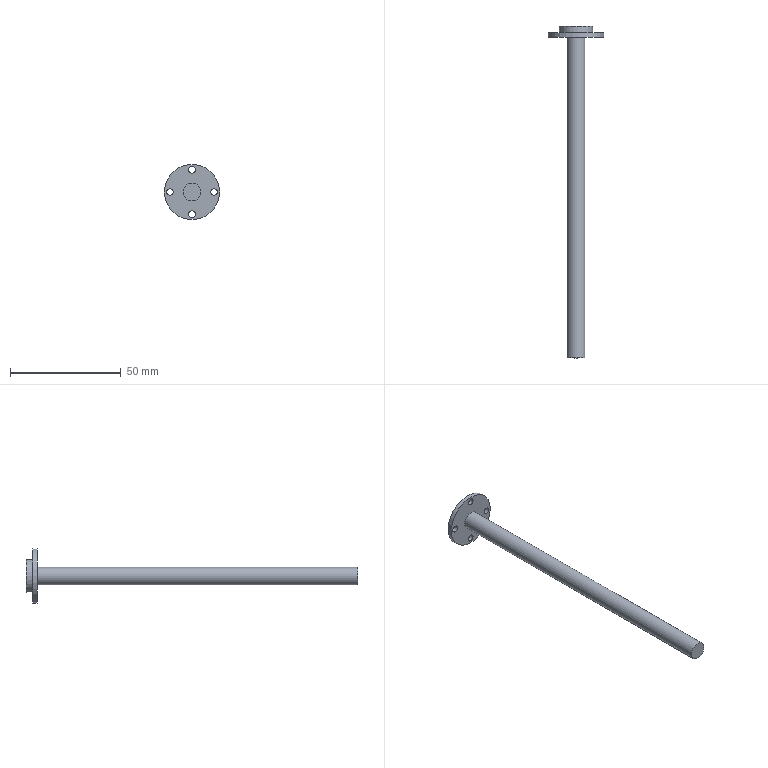Component | NX | GEAR_SHAFT_2 | 1 solid | 11 faces | box 25 x 150 x 25 mm | volume 8744 mm3 | cylinder 7 | plane 4 | commonest cylinder face diameters 3 x4 8 x1 25 x1 15 x1
STEP:
#1=CARTESIAN_POINT('',(0.,0.,0.));
#2=DIRECTION('',(0.,0.,1.));
#3=DIRECTION('',(1.,0.,0.));
#4=AXIS2_PLACEMENT_3D('',#1,#2,#3);
#5=CARTESIAN_POINT('',(-129.451,-34.96,29.835));
#6=VERTEX_POINT('',#5);
#7=CARTESIAN_POINT('',(-133.451,-34.96,29.835));
#8=DIRECTION('',(0.,1.,0.));
#9=DIRECTION('',(1.,0.,0.));
#10=AXIS2_PLACEMENT_3D('',#7,#8,#9);
#11=CIRCLE('',#10,4.);
#12=CARTESIAN_POINT('',(-133.451,-34.96,29.835));
#13=DIRECTION('',(0.,1.,0.));
#14=DIRECTION('',(0.,0.,1.));
#15=AXIS2_PLACEMENT_3D('',#12,#13,#14);
#16=CYLINDRICAL_SURFACE('',#15,4.);
#17=CARTESIAN_POINT('',(1.571,0.));
#18=DIRECTION('',(1.,0.));
#19=VECTOR('',#18,1.);
#20=LINE('',#17,#19);
#21=(GEOMETRIC_REPRESENTATION_CONTEXT(2)PARAMETRIC_REPRESENTATION_CONTEXT()REPRESENTATION_CONTEXT('',''));
#22=DEFINITIONAL_REPRESENTATION('',(#20),#21);
#23=PCURVE('',#16,#22);
#24=CARTESIAN_POINT('',(-133.451,-34.96,29.835));
#25=DIRECTION('',(0.,1.,0.));
#26=DIRECTION('',(0.,0.,1.));
#27=AXIS2_PLACEMENT_3D('',#24,#25,#26);
#28=PLANE('',#27);
#29=CARTESIAN_POINT('',(0.,0.));
#30=DIRECTION('',(0.,1.));
#31=AXIS2_PLACEMENT_2D('',#29,#30);
#32=CIRCLE('',#31,4.);
#33=(GEOMETRIC_REPRESENTATION_CONTEXT(2)PARAMETRIC_REPRESENTATION_CONTEXT()REPRESENTATION_CONTEXT('',''));
#34=DEFINITIONAL_REPRESENTATION('',(#32),#33);
#35=PCURVE('',#28,#34);
#36=SURFACE_CURVE('',#11,(#23,#35),.PCURVE_S1.);
#37=EDGE_CURVE('',#6,#6,#36,.T.);
#38=ORIENTED_EDGE('',*,*,#37,.T.);
#39=CARTESIAN_POINT('',(-129.451,110.04,29.835));
#40=VERTEX_POINT('',#39);
#41=CARTESIAN_POINT('',(-129.451,-34.96,29.835));
#42=CARTESIAN_POINT('',(-129.451,110.04,29.835));
#43=B_SPLINE_CURVE_WITH_KNOTS('',1,(#41,#42),.UNSPECIFIED.,.F.,.F.,(2,2),(0.,145.),.PIECEWISE_BEZIER_KNOTS.);
#44=CARTESIAN_POINT('',(7.854,0.));
#45=DIRECTION('',(0.,1.));
#46=VECTOR('',#45,1.);
#47=LINE('',#44,#46);
#48=(GEOMETRIC_REPRESENTATION_CONTEXT(2)PARAMETRIC_REPRESENTATION_CONTEXT()REPRESENTATION_CONTEXT('',''));
#49=DEFINITIONAL_REPRESENTATION('',(#47),#48);
#50=PCURVE('',#16,#49);
#51=CARTESIAN_POINT('',(1.571,0.));
#52=DIRECTION('',(0.,1.));
#53=VECTOR('',#52,1.);
#54=LINE('',#51,#53);
#55=(GEOMETRIC_REPRESENTATION_CONTEXT(2)PARAMETRIC_REPRESENTATION_CONTEXT()REPRESENTATION_CONTEXT('',''));
#56=DEFINITIONAL_REPRESENTATION('',(#54),#55);
#57=PCURVE('',#16,#56);
#58=SEAM_CURVE('',#43,(#50,#57),.PCURVE_S1.);
#59=EDGE_CURVE('',#6,#40,#58,.T.);
#60=ORIENTED_EDGE('',*,*,#59,.T.);
#61=CARTESIAN_POINT('',(-133.451,110.04,29.835));
#62=DIRECTION('',(0.,1.,0.));
#63=DIRECTION('',(1.,0.,0.));
#64=AXIS2_PLACEMENT_3D('',#61,#62,#63);
#65=CIRCLE('',#64,4.);
#66=CARTESIAN_POINT('',(1.571,145.));
#67=DIRECTION('',(1.,0.));
#68=VECTOR('',#67,1.);
#69=LINE('',#66,#68);
#70=(GEOMETRIC_REPRESENTATION_CONTEXT(2)PARAMETRIC_REPRESENTATION_CONTEXT()REPRESENTATION_CONTEXT('',''));
#71=DEFINITIONAL_REPRESENTATION('',(#69),#70);
#72=PCURVE('',#16,#71);
#73=CARTESIAN_POINT('',(-133.451,110.04,29.835));
#74=DIRECTION('',(0.,1.,0.));
#75=DIRECTION('',(0.,0.,1.));
#76=AXIS2_PLACEMENT_3D('',#73,#74,#75);
#77=PLANE('',#76);
#78=CARTESIAN_POINT('',(0.,0.));
#79=DIRECTION('',(0.,1.));
#80=AXIS2_PLACEMENT_2D('',#78,#79);
#81=CIRCLE('',#80,4.);
#82=(GEOMETRIC_REPRESENTATION_CONTEXT(2)PARAMETRIC_REPRESENTATION_CONTEXT()REPRESENTATION_CONTEXT('',''));
#83=DEFINITIONAL_REPRESENTATION('',(#81),#82);
#84=PCURVE('',#77,#83);
#85=SURFACE_CURVE('',#65,(#72,#84),.PCURVE_S1.);
#86=EDGE_CURVE('',#40,#40,#85,.T.);
#87=ORIENTED_EDGE('',*,*,#86,.F.);
#88=ORIENTED_EDGE('',*,*,#59,.F.);
#89=EDGE_LOOP('',(#38,#60,#87,#88));
#90=FACE_BOUND('',#89,.T.);
#91=ADVANCED_FACE('',(#90),#16,.T.);
#92=ORIENTED_EDGE('',*,*,#37,.F.);
#93=EDGE_LOOP('',(#92));
#94=FACE_BOUND('',#93,.T.);
#95=ADVANCED_FACE('',(#94),#28,.F.);
#96=CARTESIAN_POINT('',(-120.951,112.04,29.835));
#97=VERTEX_POINT('',#96);
#98=CARTESIAN_POINT('',(-133.451,112.04,29.835));
#99=DIRECTION('',(0.,-1.,0.));
#100=DIRECTION('',(1.,0.,0.));
#101=AXIS2_PLACEMENT_3D('',#98,#99,#100);
#102=CIRCLE('',#101,12.5);
#103=CARTESIAN_POINT('',(-133.451,112.04,29.835));
#104=DIRECTION('',(0.,-1.,0.));
#105=DIRECTION('',(0.,0.,-1.));
#106=AXIS2_PLACEMENT_3D('',#103,#104,#105);
#107=CYLINDRICAL_SURFACE('',#106,12.5);
#108=CARTESIAN_POINT('',(1.571,0.));
#109=DIRECTION('',(1.,0.));
#110=VECTOR('',#109,1.);
#111=LINE('',#108,#110);
#112=(GEOMETRIC_REPRESENTATION_CONTEXT(2)PARAMETRIC_REPRESENTATION_CONTEXT()REPRESENTATION_CONTEXT('',''));
#113=DEFINITIONAL_REPRESENTATION('',(#111),#112);
#114=PCURVE('',#107,#113);
#115=CARTESIAN_POINT('',(-133.451,112.04,29.835));
#116=DIRECTION('',(0.,1.,0.));
#117=DIRECTION('',(0.,0.,1.));
#118=AXIS2_PLACEMENT_3D('',#115,#116,#117);
#119=PLANE('',#118);
#120=CARTESIAN_POINT('',(0.,12.5));
#121=CARTESIAN_POINT('',(21.651,12.5));
#122=CARTESIAN_POINT('',(10.825,-6.25));
#123=CARTESIAN_POINT('',(0.,-25.));
#124=CARTESIAN_POINT('',(-10.825,-6.25));
#125=CARTESIAN_POINT('',(-21.651,12.5));
#126=CARTESIAN_POINT('',(0.,12.5));
#127=(BOUNDED_CURVE()B_SPLINE_CURVE(2,(#120,#121,#122,#123,#124,#125,#126),.UNSPECIFIED.,.T.,.F.)B_SPLINE_CURVE_WITH_KNOTS((1,2,2,2,2,1),(-2.094,0.,2.094,4.189,6.283,8.378),.UNSPECIFIED.)CURVE()GEOMETRIC_REPRESENTATION_ITEM()RATIONAL_B_SPLINE_CURVE((1.,0.5,1.,0.5,1.,0.5,1.))REPRESENTATION_ITEM(''));
#128=(GEOMETRIC_REPRESENTATION_CONTEXT(2)PARAMETRIC_REPRESENTATION_CONTEXT()REPRESENTATION_CONTEXT('',''));
#129=DEFINITIONAL_REPRESENTATION('',(#127),#128);
#130=PCURVE('',#119,#129);
#131=SURFACE_CURVE('',#102,(#114,#130),.PCURVE_S1.);
#132=EDGE_CURVE('',#97,#97,#131,.T.);
#133=ORIENTED_EDGE('',*,*,#132,.T.);
#134=CARTESIAN_POINT('',(-120.951,110.04,29.835));
#135=VERTEX_POINT('',#134);
#136=CARTESIAN_POINT('',(-120.951,112.04,29.835));
#137=CARTESIAN_POINT('',(-120.951,110.04,29.835));
#138=B_SPLINE_CURVE_WITH_KNOTS('',1,(#136,#137),.UNSPECIFIED.,.F.,.F.,(2,2),(0.,2.),.PIECEWISE_BEZIER_KNOTS.);
#139=CARTESIAN_POINT('',(7.854,0.));
#140=DIRECTION('',(0.,1.));
#141=VECTOR('',#140,1.);
#142=LINE('',#139,#141);
#143=(GEOMETRIC_REPRESENTATION_CONTEXT(2)PARAMETRIC_REPRESENTATION_CONTEXT()REPRESENTATION_CONTEXT('',''));
#144=DEFINITIONAL_REPRESENTATION('',(#142),#143);
#145=PCURVE('',#107,#144);
#146=CARTESIAN_POINT('',(1.571,0.));
#147=DIRECTION('',(0.,1.));
#148=VECTOR('',#147,1.);
#149=LINE('',#146,#148);
#150=(GEOMETRIC_REPRESENTATION_CONTEXT(2)PARAMETRIC_REPRESENTATION_CONTEXT()REPRESENTATION_CONTEXT('',''));
#151=DEFINITIONAL_REPRESENTATION('',(#149),#150);
#152=PCURVE('',#107,#151);
#153=SEAM_CURVE('',#138,(#145,#152),.PCURVE_S1.);
#154=EDGE_CURVE('',#97,#135,#153,.T.);
#155=ORIENTED_EDGE('',*,*,#154,.T.);
#156=CARTESIAN_POINT('',(-133.451,110.04,29.835));
#157=DIRECTION('',(0.,-1.,0.));
#158=DIRECTION('',(1.,0.,0.));
#159=AXIS2_PLACEMENT_3D('',#156,#157,#158);
#160=CIRCLE('',#159,12.5);
#161=CARTESIAN_POINT('',(1.571,2.));
#162=DIRECTION('',(1.,0.));
#163=VECTOR('',#162,1.);
#164=LINE('',#161,#163);
#165=(GEOMETRIC_REPRESENTATION_CONTEXT(2)PARAMETRIC_REPRESENTATION_CONTEXT()REPRESENTATION_CONTEXT('',''));
#166=DEFINITIONAL_REPRESENTATION('',(#164),#165);
#167=PCURVE('',#107,#166);
#168=CARTESIAN_POINT('',(0.,12.5));
#169=CARTESIAN_POINT('',(21.651,12.5));
#170=CARTESIAN_POINT('',(10.825,-6.25));
#171=CARTESIAN_POINT('',(0.,-25.));
#172=CARTESIAN_POINT('',(-10.825,-6.25));
#173=CARTESIAN_POINT('',(-21.651,12.5));
#174=CARTESIAN_POINT('',(0.,12.5));
#175=(BOUNDED_CURVE()B_SPLINE_CURVE(2,(#168,#169,#170,#171,#172,#173,#174),.UNSPECIFIED.,.T.,.F.)B_SPLINE_CURVE_WITH_KNOTS((1,2,2,2,2,1),(-2.094,0.,2.094,4.189,6.283,8.378),.UNSPECIFIED.)CURVE()GEOMETRIC_REPRESENTATION_ITEM()RATIONAL_B_SPLINE_CURVE((1.,0.5,1.,0.5,1.,0.5,1.))REPRESENTATION_ITEM(''));
#176=(GEOMETRIC_REPRESENTATION_CONTEXT(2)PARAMETRIC_REPRESENTATION_CONTEXT()REPRESENTATION_CONTEXT('',''));
#177=DEFINITIONAL_REPRESENTATION('',(#175),#176);
#178=PCURVE('',#77,#177);
#179=SURFACE_CURVE('',#160,(#167,#178),.PCURVE_S1.);
#180=EDGE_CURVE('',#135,#135,#179,.T.);
#181=ORIENTED_EDGE('',*,*,#180,.F.);
#182=ORIENTED_EDGE('',*,*,#154,.F.);
#183=EDGE_LOOP('',(#133,#155,#181,#182));
#184=FACE_BOUND('',#183,.T.);
#185=ADVANCED_FACE('',(#184),#107,.T.);
#186=CARTESIAN_POINT('',(-133.451,112.04,18.335));
#187=VERTEX_POINT('',#186);
#188=CARTESIAN_POINT('',(-133.451,112.04,21.335));
#189=VERTEX_POINT('',#188);
#190=CARTESIAN_POINT('',(-133.451,112.04,19.835));
#191=DIRECTION('',(0.,-1.,0.));
#192=DIRECTION('',(0.,0.,-1.));
#193=AXIS2_PLACEMENT_3D('',#190,#191,#192);
#194=CIRCLE('',#193,1.5);
#195=CARTESIAN_POINT('',(-11.5,0.));
#196=CARTESIAN_POINT('',(-11.5,2.598));
#197=CARTESIAN_POINT('',(-9.25,1.299));
#198=CARTESIAN_POINT('',(-7.,0.));
#199=CARTESIAN_POINT('',(-9.25,-1.299));
#200=CARTESIAN_POINT('',(-11.5,-2.598));
#201=CARTESIAN_POINT('',(-11.5,0.));
#202=(BOUNDED_CURVE()B_SPLINE_CURVE(2,(#195,#196,#197,#198,#199,#200,#201),.UNSPECIFIED.,.T.,.F.)B_SPLINE_CURVE_WITH_KNOTS((1,2,2,2,2,1),(-2.094,0.,2.094,4.189,6.283,8.378),.UNSPECIFIED.)CURVE()GEOMETRIC_REPRESENTATION_ITEM()RATIONAL_B_SPLINE_CURVE((1.,0.5,1.,0.5,1.,0.5,1.))REPRESENTATION_ITEM(''));
#203=(GEOMETRIC_REPRESENTATION_CONTEXT(2)PARAMETRIC_REPRESENTATION_CONTEXT()REPRESENTATION_CONTEXT('',''));
#204=DEFINITIONAL_REPRESENTATION('',(#202),#203);
#205=PCURVE('',#119,#204);
#206=CARTESIAN_POINT('',(-133.451,-87.96,19.835));
#207=DIRECTION('',(0.,1.,0.));
#208=DIRECTION('',(0.,0.,1.));
#209=AXIS2_PLACEMENT_3D('',#206,#207,#208);
#210=CYLINDRICAL_SURFACE('',#209,1.5);
#211=CARTESIAN_POINT('',(3.142,200.));
#212=DIRECTION('',(-1.,0.));
#213=VECTOR('',#212,1.);
#214=LINE('',#211,#213);
#215=(GEOMETRIC_REPRESENTATION_CONTEXT(2)PARAMETRIC_REPRESENTATION_CONTEXT()REPRESENTATION_CONTEXT('',''));
#216=DEFINITIONAL_REPRESENTATION('',(#214),#215);
#217=PCURVE('',#210,#216);
#218=SURFACE_CURVE('',#194,(#205,#217),.PCURVE_S1.);
#219=EDGE_CURVE('',#187,#189,#218,.T.);
#220=ORIENTED_EDGE('',*,*,#219,.T.);
#221=CARTESIAN_POINT('',(-133.451,112.04,19.835));
#222=DIRECTION('',(0.,-1.,0.));
#223=DIRECTION('',(0.,0.,-1.));
#224=AXIS2_PLACEMENT_3D('',#221,#222,#223);
#225=CIRCLE('',#224,1.5);
#226=CARTESIAN_POINT('',(-11.5,0.));
#227=CARTESIAN_POINT('',(-11.5,2.598));
#228=CARTESIAN_POINT('',(-9.25,1.299));
#229=CARTESIAN_POINT('',(-7.,0.));
#230=CARTESIAN_POINT('',(-9.25,-1.299));
#231=CARTESIAN_POINT('',(-11.5,-2.598));
#232=CARTESIAN_POINT('',(-11.5,0.));
#233=(BOUNDED_CURVE()B_SPLINE_CURVE(2,(#226,#227,#228,#229,#230,#231,#232),.UNSPECIFIED.,.T.,.F.)B_SPLINE_CURVE_WITH_KNOTS((1,2,2,2,2,1),(-2.094,0.,2.094,4.189,6.283,8.378),.UNSPECIFIED.)CURVE()GEOMETRIC_REPRESENTATION_ITEM()RATIONAL_B_SPLINE_CURVE((1.,0.5,1.,0.5,1.,0.5,1.))REPRESENTATION_ITEM(''));
#234=(GEOMETRIC_REPRESENTATION_CONTEXT(2)PARAMETRIC_REPRESENTATION_CONTEXT()REPRESENTATION_CONTEXT('',''));
#235=DEFINITIONAL_REPRESENTATION('',(#233),#234);
#236=PCURVE('',#119,#235);
#237=CARTESIAN_POINT('',(9.425,200.));
#238=DIRECTION('',(-1.,0.));
#239=VECTOR('',#238,1.);
#240=LINE('',#237,#239);
#241=(GEOMETRIC_REPRESENTATION_CONTEXT(2)PARAMETRIC_REPRESENTATION_CONTEXT()REPRESENTATION_CONTEXT('',''));
#242=DEFINITIONAL_REPRESENTATION('',(#240),#241);
#243=PCURVE('',#210,#242);
#244=SURFACE_CURVE('',#225,(#236,#243),.PCURVE_S1.);
#245=EDGE_CURVE('',#189,#187,#244,.T.);
#246=ORIENTED_EDGE('',*,*,#245,.T.);
#247=EDGE_LOOP('',(#220,#246));
#248=FACE_BOUND('',#247,.T.);
#249=CARTESIAN_POINT('',(-144.951,112.04,29.835));
#250=VERTEX_POINT('',#249);
#251=CARTESIAN_POINT('',(-143.451,112.04,31.335));
#252=VERTEX_POINT('',#251);
#253=CARTESIAN_POINT('',(-143.451,112.04,29.835));
#254=DIRECTION('',(0.,1.,0.));
#255=DIRECTION('',(-1.,0.,0.));
#256=AXIS2_PLACEMENT_3D('',#253,#254,#255);
#257=CIRCLE('',#256,1.5);
#258=CARTESIAN_POINT('',(0.,-10.));
#259=DIRECTION('',(0.,-1.));
#260=AXIS2_PLACEMENT_2D('',#258,#259);
#261=CIRCLE('',#260,1.5);
#262=(GEOMETRIC_REPRESENTATION_CONTEXT(2)PARAMETRIC_REPRESENTATION_CONTEXT()REPRESENTATION_CONTEXT('',''));
#263=DEFINITIONAL_REPRESENTATION('',(#261),#262);
#264=PCURVE('',#119,#263);
#265=CARTESIAN_POINT('',(-143.451,-87.96,29.835));
#266=DIRECTION('',(0.,1.,0.));
#267=DIRECTION('',(0.,0.,1.));
#268=AXIS2_PLACEMENT_3D('',#265,#266,#267);
#269=CYLINDRICAL_SURFACE('',#268,1.5);
#270=CARTESIAN_POINT('',(4.712,200.));
#271=DIRECTION('',(1.,0.));
#272=VECTOR('',#271,1.);
#273=LINE('',#270,#272);
#274=(GEOMETRIC_REPRESENTATION_CONTEXT(2)PARAMETRIC_REPRESENTATION_CONTEXT()REPRESENTATION_CONTEXT('',''));
#275=DEFINITIONAL_REPRESENTATION('',(#273),#274);
#276=PCURVE('',#269,#275);
#277=SURFACE_CURVE('',#257,(#264,#276),.PCURVE_S1.);
#278=EDGE_CURVE('',#250,#252,#277,.T.);
#279=ORIENTED_EDGE('',*,*,#278,.F.);
#280=CARTESIAN_POINT('',(-143.451,112.04,29.835));
#281=DIRECTION('',(0.,1.,0.));
#282=DIRECTION('',(-1.,0.,0.));
#283=AXIS2_PLACEMENT_3D('',#280,#281,#282);
#284=CIRCLE('',#283,1.5);
#285=CARTESIAN_POINT('',(0.,-10.));
#286=DIRECTION('',(0.,-1.));
#287=AXIS2_PLACEMENT_2D('',#285,#286);
#288=CIRCLE('',#287,1.5);
#289=(GEOMETRIC_REPRESENTATION_CONTEXT(2)PARAMETRIC_REPRESENTATION_CONTEXT()REPRESENTATION_CONTEXT('',''));
#290=DEFINITIONAL_REPRESENTATION('',(#288),#289);
#291=PCURVE('',#119,#290);
#292=CARTESIAN_POINT('',(-1.571,200.));
#293=DIRECTION('',(1.,0.));
#294=VECTOR('',#293,1.);
#295=LINE('',#292,#294);
#296=(GEOMETRIC_REPRESENTATION_CONTEXT(2)PARAMETRIC_REPRESENTATION_CONTEXT()REPRESENTATION_CONTEXT('',''));
#297=DEFINITIONAL_REPRESENTATION('',(#295),#296);
#298=PCURVE('',#269,#297);
#299=SURFACE_CURVE('',#284,(#291,#298),.PCURVE_S1.);
#300=EDGE_CURVE('',#252,#250,#299,.T.);
#301=ORIENTED_EDGE('',*,*,#300,.F.);
#302=EDGE_LOOP('',(#279,#301));
#303=FACE_BOUND('',#302,.T.);
#304=CARTESIAN_POINT('',(-133.451,112.04,41.335));
#305=VERTEX_POINT('',#304);
#306=CARTESIAN_POINT('',(-133.451,112.04,39.835));
#307=DIRECTION('',(0.,1.,0.));
#308=DIRECTION('',(0.,0.,1.));
#309=AXIS2_PLACEMENT_3D('',#306,#307,#308);
#310=CIRCLE('',#309,1.5);
#311=CARTESIAN_POINT('',(10.,0.));
#312=DIRECTION('',(1.,0.));
#313=AXIS2_PLACEMENT_2D('',#311,#312);
#314=CIRCLE('',#313,1.5);
#315=(GEOMETRIC_REPRESENTATION_CONTEXT(2)PARAMETRIC_REPRESENTATION_CONTEXT()REPRESENTATION_CONTEXT('',''));
#316=DEFINITIONAL_REPRESENTATION('',(#314),#315);
#317=PCURVE('',#119,#316);
#318=CARTESIAN_POINT('',(-133.451,-87.96,39.835));
#319=DIRECTION('',(0.,1.,0.));
#320=DIRECTION('',(0.,0.,1.));
#321=AXIS2_PLACEMENT_3D('',#318,#319,#320);
#322=CYLINDRICAL_SURFACE('',#321,1.5);
#323=CARTESIAN_POINT('',(0.,200.));
#324=DIRECTION('',(1.,0.));
#325=VECTOR('',#324,1.);
#326=LINE('',#323,#325);
#327=(GEOMETRIC_REPRESENTATION_CONTEXT(2)PARAMETRIC_REPRESENTATION_CONTEXT()REPRESENTATION_CONTEXT('',''));
#328=DEFINITIONAL_REPRESENTATION('',(#326),#327);
#329=PCURVE('',#322,#328);
#330=SURFACE_CURVE('',#310,(#317,#329),.PCURVE_S1.);
#331=EDGE_CURVE('',#305,#305,#330,.T.);
#332=ORIENTED_EDGE('',*,*,#331,.F.);
#333=EDGE_LOOP('',(#332));
#334=FACE_BOUND('',#333,.T.);
#335=CARTESIAN_POINT('',(-121.951,112.04,29.835));
#336=VERTEX_POINT('',#335);
#337=CARTESIAN_POINT('',(-123.451,112.04,31.335));
#338=VERTEX_POINT('',#337);
#339=CARTESIAN_POINT('',(-123.451,112.04,29.835));
#340=DIRECTION('',(0.,1.,0.));
#341=DIRECTION('',(1.,0.,0.));
#342=AXIS2_PLACEMENT_3D('',#339,#340,#341);
#343=CIRCLE('',#342,1.5);
#344=CARTESIAN_POINT('',(0.,10.));
#345=DIRECTION('',(0.,1.));
#346=AXIS2_PLACEMENT_2D('',#344,#345);
#347=CIRCLE('',#346,1.5);
#348=(GEOMETRIC_REPRESENTATION_CONTEXT(2)PARAMETRIC_REPRESENTATION_CONTEXT()REPRESENTATION_CONTEXT('',''));
#349=DEFINITIONAL_REPRESENTATION('',(#347),#348);
#350=PCURVE('',#119,#349);
#351=CARTESIAN_POINT('',(-123.451,-87.96,29.835));
#352=DIRECTION('',(0.,1.,0.));
#353=DIRECTION('',(0.,0.,1.));
#354=AXIS2_PLACEMENT_3D('',#351,#352,#353);
#355=CYLINDRICAL_SURFACE('',#354,1.5);
#356=CARTESIAN_POINT('',(1.571,200.));
#357=DIRECTION('',(1.,0.));
#358=VECTOR('',#357,1.);
#359=LINE('',#356,#358);
#360=(GEOMETRIC_REPRESENTATION_CONTEXT(2)PARAMETRIC_REPRESENTATION_CONTEXT()REPRESENTATION_CONTEXT('',''));
#361=DEFINITIONAL_REPRESENTATION('',(#359),#360);
#362=PCURVE('',#355,#361);
#363=SURFACE_CURVE('',#343,(#350,#362),.PCURVE_S1.);
#364=EDGE_CURVE('',#336,#338,#363,.T.);
#365=ORIENTED_EDGE('',*,*,#364,.F.);
#366=CARTESIAN_POINT('',(-123.451,112.04,29.835));
#367=DIRECTION('',(0.,1.,0.));
#368=DIRECTION('',(1.,0.,0.));
#369=AXIS2_PLACEMENT_3D('',#366,#367,#368);
#370=CIRCLE('',#369,1.5);
#371=CARTESIAN_POINT('',(0.,10.));
#372=DIRECTION('',(0.,1.));
#373=AXIS2_PLACEMENT_2D('',#371,#372);
#374=CIRCLE('',#373,1.5);
#375=(GEOMETRIC_REPRESENTATION_CONTEXT(2)PARAMETRIC_REPRESENTATION_CONTEXT()REPRESENTATION_CONTEXT('',''));
#376=DEFINITIONAL_REPRESENTATION('',(#374),#375);
#377=PCURVE('',#119,#376);
#378=CARTESIAN_POINT('',(-4.712,200.));
#379=DIRECTION('',(1.,0.));
#380=VECTOR('',#379,1.);
#381=LINE('',#378,#380);
#382=(GEOMETRIC_REPRESENTATION_CONTEXT(2)PARAMETRIC_REPRESENTATION_CONTEXT()REPRESENTATION_CONTEXT('',''));
#383=DEFINITIONAL_REPRESENTATION('',(#381),#382);
#384=PCURVE('',#355,#383);
#385=SURFACE_CURVE('',#370,(#377,#384),.PCURVE_S1.);
#386=EDGE_CURVE('',#338,#336,#385,.T.);
#387=ORIENTED_EDGE('',*,*,#386,.F.);
#388=EDGE_LOOP('',(#365,#387));
#389=FACE_BOUND('',#388,.T.);
#390=CARTESIAN_POINT('',(-125.951,112.04,29.835));
#391=VERTEX_POINT('',#390);
#392=CARTESIAN_POINT('',(-133.451,112.04,29.835));
#393=DIRECTION('',(0.,1.,0.));
#394=DIRECTION('',(1.,0.,0.));
#395=AXIS2_PLACEMENT_3D('',#392,#393,#394);
#396=CIRCLE('',#395,7.5);
#397=CARTESIAN_POINT('',(0.,0.));
#398=DIRECTION('',(0.,1.));
#399=AXIS2_PLACEMENT_2D('',#397,#398);
#400=CIRCLE('',#399,7.5);
#401=(GEOMETRIC_REPRESENTATION_CONTEXT(2)PARAMETRIC_REPRESENTATION_CONTEXT()REPRESENTATION_CONTEXT('',''));
#402=DEFINITIONAL_REPRESENTATION('',(#400),#401);
#403=PCURVE('',#119,#402);
#404=CARTESIAN_POINT('',(-133.451,115.04,29.835));
#405=DIRECTION('',(0.,-1.,0.));
#406=DIRECTION('',(0.,0.,-1.));
#407=AXIS2_PLACEMENT_3D('',#404,#405,#406);
#408=CYLINDRICAL_SURFACE('',#407,7.5);
#409=CARTESIAN_POINT('',(7.854,3.));
#410=DIRECTION('',(-1.,0.));
#411=VECTOR('',#410,1.);
#412=LINE('',#409,#411);
#413=(GEOMETRIC_REPRESENTATION_CONTEXT(2)PARAMETRIC_REPRESENTATION_CONTEXT()REPRESENTATION_CONTEXT('',''));
#414=DEFINITIONAL_REPRESENTATION('',(#412),#413);
#415=PCURVE('',#408,#414);
#416=SURFACE_CURVE('',#396,(#403,#415),.PCURVE_S1.);
#417=EDGE_CURVE('',#391,#391,#416,.T.);
#418=ORIENTED_EDGE('',*,*,#417,.F.);
#419=EDGE_LOOP('',(#418));
#420=FACE_BOUND('',#419,.T.);
#421=ORIENTED_EDGE('',*,*,#132,.F.);
#422=EDGE_LOOP('',(#421));
#423=FACE_BOUND('',#422,.T.);
#424=ADVANCED_FACE('',(#248,#303,#334,#389,#420,#423),#119,.T.);
#425=CARTESIAN_POINT('',(-133.451,110.04,21.335));
#426=VERTEX_POINT('',#425);
#427=CARTESIAN_POINT('',(-133.451,110.04,19.835));
#428=DIRECTION('',(0.,-1.,0.));
#429=DIRECTION('',(0.,0.,1.));
#430=AXIS2_PLACEMENT_3D('',#427,#428,#429);
#431=CIRCLE('',#430,1.5);
#432=CARTESIAN_POINT('',(-8.5,0.));
#433=CARTESIAN_POINT('',(-8.5,-2.598));
#434=CARTESIAN_POINT('',(-10.75,-1.299));
#435=CARTESIAN_POINT('',(-13.,-0.));
#436=CARTESIAN_POINT('',(-10.75,1.299));
#437=CARTESIAN_POINT('',(-8.5,2.598));
#438=CARTESIAN_POINT('',(-8.5,0.));
#439=(BOUNDED_CURVE()B_SPLINE_CURVE(2,(#432,#433,#434,#435,#436,#437,#438),.UNSPECIFIED.,.T.,.F.)B_SPLINE_CURVE_WITH_KNOTS((1,2,2,2,2,1),(-2.094,0.,2.094,4.189,6.283,8.378),.UNSPECIFIED.)CURVE()GEOMETRIC_REPRESENTATION_ITEM()RATIONAL_B_SPLINE_CURVE((1.,0.5,1.,0.5,1.,0.5,1.))REPRESENTATION_ITEM(''));
#440=(GEOMETRIC_REPRESENTATION_CONTEXT(2)PARAMETRIC_REPRESENTATION_CONTEXT()REPRESENTATION_CONTEXT('',''));
#441=DEFINITIONAL_REPRESENTATION('',(#439),#440);
#442=PCURVE('',#77,#441);
#443=CARTESIAN_POINT('',(6.283,198.));
#444=DIRECTION('',(-1.,0.));
#445=VECTOR('',#444,1.);
#446=LINE('',#443,#445);
#447=(GEOMETRIC_REPRESENTATION_CONTEXT(2)PARAMETRIC_REPRESENTATION_CONTEXT()REPRESENTATION_CONTEXT('',''));
#448=DEFINITIONAL_REPRESENTATION('',(#446),#447);
#449=PCURVE('',#210,#448);
#450=SURFACE_CURVE('',#431,(#442,#449),.PCURVE_S1.);
#451=EDGE_CURVE('',#426,#426,#450,.T.);
#452=ORIENTED_EDGE('',*,*,#451,.F.);
#453=EDGE_LOOP('',(#452));
#454=FACE_BOUND('',#453,.T.);
#455=CARTESIAN_POINT('',(-143.451,110.04,31.335));
#456=VERTEX_POINT('',#455);
#457=CARTESIAN_POINT('',(-143.451,110.04,29.835));
#458=DIRECTION('',(0.,1.,0.));
#459=DIRECTION('',(0.,0.,1.));
#460=AXIS2_PLACEMENT_3D('',#457,#458,#459);
#461=CIRCLE('',#460,1.5);
#462=CARTESIAN_POINT('',(0.,-10.));
#463=DIRECTION('',(1.,0.));
#464=AXIS2_PLACEMENT_2D('',#462,#463);
#465=CIRCLE('',#464,1.5);
#466=(GEOMETRIC_REPRESENTATION_CONTEXT(2)PARAMETRIC_REPRESENTATION_CONTEXT()REPRESENTATION_CONTEXT('',''));
#467=DEFINITIONAL_REPRESENTATION('',(#465),#466);
#468=PCURVE('',#77,#467);
#469=CARTESIAN_POINT('',(0.,198.));
#470=DIRECTION('',(1.,0.));
#471=VECTOR('',#470,1.);
#472=LINE('',#469,#471);
#473=(GEOMETRIC_REPRESENTATION_CONTEXT(2)PARAMETRIC_REPRESENTATION_CONTEXT()REPRESENTATION_CONTEXT('',''));
#474=DEFINITIONAL_REPRESENTATION('',(#472),#473);
#475=PCURVE('',#269,#474);
#476=SURFACE_CURVE('',#461,(#468,#475),.PCURVE_S1.);
#477=EDGE_CURVE('',#456,#456,#476,.T.);
#478=ORIENTED_EDGE('',*,*,#477,.T.);
#479=EDGE_LOOP('',(#478));
#480=FACE_BOUND('',#479,.T.);
#481=CARTESIAN_POINT('',(-133.451,110.04,41.335));
#482=VERTEX_POINT('',#481);
#483=CARTESIAN_POINT('',(-133.451,110.04,39.835));
#484=DIRECTION('',(0.,1.,0.));
#485=DIRECTION('',(0.,0.,1.));
#486=AXIS2_PLACEMENT_3D('',#483,#484,#485);
#487=CIRCLE('',#486,1.5);
#488=CARTESIAN_POINT('',(10.,0.));
#489=DIRECTION('',(1.,0.));
#490=AXIS2_PLACEMENT_2D('',#488,#489);
#491=CIRCLE('',#490,1.5);
#492=(GEOMETRIC_REPRESENTATION_CONTEXT(2)PARAMETRIC_REPRESENTATION_CONTEXT()REPRESENTATION_CONTEXT('',''));
#493=DEFINITIONAL_REPRESENTATION('',(#491),#492);
#494=PCURVE('',#77,#493);
#495=CARTESIAN_POINT('',(0.,198.));
#496=DIRECTION('',(1.,0.));
#497=VECTOR('',#496,1.);
#498=LINE('',#495,#497);
#499=(GEOMETRIC_REPRESENTATION_CONTEXT(2)PARAMETRIC_REPRESENTATION_CONTEXT()REPRESENTATION_CONTEXT('',''));
#500=DEFINITIONAL_REPRESENTATION('',(#498),#499);
#501=PCURVE('',#322,#500);
#502=SURFACE_CURVE('',#487,(#494,#501),.PCURVE_S1.);
#503=EDGE_CURVE('',#482,#482,#502,.T.);
#504=ORIENTED_EDGE('',*,*,#503,.T.);
#505=EDGE_LOOP('',(#504));
#506=FACE_BOUND('',#505,.T.);
#507=CARTESIAN_POINT('',(-123.451,110.04,31.335));
#508=VERTEX_POINT('',#507);
#509=CARTESIAN_POINT('',(-123.451,110.04,29.835));
#510=DIRECTION('',(0.,1.,0.));
#511=DIRECTION('',(0.,0.,1.));
#512=AXIS2_PLACEMENT_3D('',#509,#510,#511);
#513=CIRCLE('',#512,1.5);
#514=CARTESIAN_POINT('',(0.,10.));
#515=DIRECTION('',(1.,0.));
#516=AXIS2_PLACEMENT_2D('',#514,#515);
#517=CIRCLE('',#516,1.5);
#518=(GEOMETRIC_REPRESENTATION_CONTEXT(2)PARAMETRIC_REPRESENTATION_CONTEXT()REPRESENTATION_CONTEXT('',''));
#519=DEFINITIONAL_REPRESENTATION('',(#517),#518);
#520=PCURVE('',#77,#519);
#521=CARTESIAN_POINT('',(0.,198.));
#522=DIRECTION('',(1.,0.));
#523=VECTOR('',#522,1.);
#524=LINE('',#521,#523);
#525=(GEOMETRIC_REPRESENTATION_CONTEXT(2)PARAMETRIC_REPRESENTATION_CONTEXT()REPRESENTATION_CONTEXT('',''));
#526=DEFINITIONAL_REPRESENTATION('',(#524),#525);
#527=PCURVE('',#355,#526);
#528=SURFACE_CURVE('',#513,(#520,#527),.PCURVE_S1.);
#529=EDGE_CURVE('',#508,#508,#528,.T.);
#530=ORIENTED_EDGE('',*,*,#529,.T.);
#531=EDGE_LOOP('',(#530));
#532=FACE_BOUND('',#531,.T.);
#533=ORIENTED_EDGE('',*,*,#86,.T.);
#534=EDGE_LOOP('',(#533));
#535=FACE_BOUND('',#534,.T.);
#536=ORIENTED_EDGE('',*,*,#180,.T.);
#537=EDGE_LOOP('',(#536));
#538=FACE_BOUND('',#537,.T.);
#539=ADVANCED_FACE('',(#454,#480,#506,#532,#535,#538),#77,.F.);
#540=CARTESIAN_POINT('',(-125.951,115.04,29.835));
#541=VERTEX_POINT('',#540);
#542=CARTESIAN_POINT('',(-133.451,115.04,29.835));
#543=DIRECTION('',(0.,1.,0.));
#544=DIRECTION('',(1.,0.,0.));
#545=AXIS2_PLACEMENT_3D('',#542,#543,#544);
#546=CIRCLE('',#545,7.5);
#547=CARTESIAN_POINT('',(7.854,0.));
#548=DIRECTION('',(-1.,0.));
#549=VECTOR('',#548,1.);
#550=LINE('',#547,#549);
#551=(GEOMETRIC_REPRESENTATION_CONTEXT(2)PARAMETRIC_REPRESENTATION_CONTEXT()REPRESENTATION_CONTEXT('',''));
#552=DEFINITIONAL_REPRESENTATION('',(#550),#551);
#553=PCURVE('',#408,#552);
#554=CARTESIAN_POINT('',(-133.451,115.04,29.835));
#555=DIRECTION('',(0.,1.,0.));
#556=DIRECTION('',(0.,0.,1.));
#557=AXIS2_PLACEMENT_3D('',#554,#555,#556);
#558=PLANE('',#557);
#559=CARTESIAN_POINT('',(0.,0.));
#560=DIRECTION('',(0.,1.));
#561=AXIS2_PLACEMENT_2D('',#559,#560);
#562=CIRCLE('',#561,7.5);
#563=(GEOMETRIC_REPRESENTATION_CONTEXT(2)PARAMETRIC_REPRESENTATION_CONTEXT()REPRESENTATION_CONTEXT('',''));
#564=DEFINITIONAL_REPRESENTATION('',(#562),#563);
#565=PCURVE('',#558,#564);
#566=SURFACE_CURVE('',#546,(#553,#565),.PCURVE_S1.);
#567=EDGE_CURVE('',#541,#541,#566,.T.);
#568=ORIENTED_EDGE('',*,*,#567,.F.);
#569=CARTESIAN_POINT('',(-125.951,115.04,29.835));
#570=CARTESIAN_POINT('',(-125.951,112.04,29.835));
#571=B_SPLINE_CURVE_WITH_KNOTS('',1,(#569,#570),.UNSPECIFIED.,.F.,.F.,(2,2),(0.,3.),.PIECEWISE_BEZIER_KNOTS.);
#572=CARTESIAN_POINT('',(7.854,0.));
#573=DIRECTION('',(0.,1.));
#574=VECTOR('',#573,1.);
#575=LINE('',#572,#574);
#576=(GEOMETRIC_REPRESENTATION_CONTEXT(2)PARAMETRIC_REPRESENTATION_CONTEXT()REPRESENTATION_CONTEXT('',''));
#577=DEFINITIONAL_REPRESENTATION('',(#575),#576);
#578=PCURVE('',#408,#577);
#579=CARTESIAN_POINT('',(1.571,0.));
#580=DIRECTION('',(0.,1.));
#581=VECTOR('',#580,1.);
#582=LINE('',#579,#581);
#583=(GEOMETRIC_REPRESENTATION_CONTEXT(2)PARAMETRIC_REPRESENTATION_CONTEXT()REPRESENTATION_CONTEXT('',''));
#584=DEFINITIONAL_REPRESENTATION('',(#582),#583);
#585=PCURVE('',#408,#584);
#586=SEAM_CURVE('',#571,(#578,#585),.PCURVE_S1.);
#587=EDGE_CURVE('',#541,#391,#586,.T.);
#588=ORIENTED_EDGE('',*,*,#587,.T.);
#589=ORIENTED_EDGE('',*,*,#417,.T.);
#590=ORIENTED_EDGE('',*,*,#587,.F.);
#591=EDGE_LOOP('',(#568,#588,#589,#590));
#592=FACE_BOUND('',#591,.T.);
#593=ADVANCED_FACE('',(#592),#408,.T.);
#594=ORIENTED_EDGE('',*,*,#567,.T.);
#595=EDGE_LOOP('',(#594));
#596=FACE_BOUND('',#595,.T.);
#597=ADVANCED_FACE('',(#596),#558,.T.);
#598=ORIENTED_EDGE('',*,*,#386,.F.);
#599=CARTESIAN_POINT('',(-123.451,110.04,31.335));
#600=CARTESIAN_POINT('',(-123.451,112.04,31.335));
#601=B_SPLINE_CURVE_WITH_KNOTS('',1,(#599,#600),.UNSPECIFIED.,.F.,.F.,(2,2),(198.,200.),.PIECEWISE_BEZIER_KNOTS.);
#602=CARTESIAN_POINT('',(0.,0.));
#603=DIRECTION('',(0.,1.));
#604=VECTOR('',#603,1.);
#605=LINE('',#602,#604);
#606=(GEOMETRIC_REPRESENTATION_CONTEXT(2)PARAMETRIC_REPRESENTATION_CONTEXT()REPRESENTATION_CONTEXT('',''));
#607=DEFINITIONAL_REPRESENTATION('',(#605),#606);
#608=PCURVE('',#355,#607);
#609=CARTESIAN_POINT('',(6.283,0.));
#610=DIRECTION('',(0.,1.));
#611=VECTOR('',#610,1.);
#612=LINE('',#609,#611);
#613=(GEOMETRIC_REPRESENTATION_CONTEXT(2)PARAMETRIC_REPRESENTATION_CONTEXT()REPRESENTATION_CONTEXT('',''));
#614=DEFINITIONAL_REPRESENTATION('',(#612),#613);
#615=PCURVE('',#355,#614);
#616=SEAM_CURVE('',#601,(#608,#615),.PCURVE_S1.);
#617=EDGE_CURVE('',#508,#338,#616,.T.);
#618=ORIENTED_EDGE('',*,*,#617,.F.);
#619=ORIENTED_EDGE('',*,*,#529,.T.);
#620=ORIENTED_EDGE('',*,*,#617,.T.);
#621=ORIENTED_EDGE('',*,*,#364,.F.);
#622=EDGE_LOOP('',(#598,#618,#619,#620,#621));
#623=FACE_BOUND('',#622,.F.);
#624=ADVANCED_FACE('',(#623),#355,.F.);
#625=ORIENTED_EDGE('',*,*,#331,.F.);
#626=CARTESIAN_POINT('',(-133.451,110.04,41.335));
#627=CARTESIAN_POINT('',(-133.451,112.04,41.335));
#628=B_SPLINE_CURVE_WITH_KNOTS('',1,(#626,#627),.UNSPECIFIED.,.F.,.F.,(2,2),(198.,200.),.PIECEWISE_BEZIER_KNOTS.);
#629=CARTESIAN_POINT('',(0.,0.));
#630=DIRECTION('',(0.,1.));
#631=VECTOR('',#630,1.);
#632=LINE('',#629,#631);
#633=(GEOMETRIC_REPRESENTATION_CONTEXT(2)PARAMETRIC_REPRESENTATION_CONTEXT()REPRESENTATION_CONTEXT('',''));
#634=DEFINITIONAL_REPRESENTATION('',(#632),#633);
#635=PCURVE('',#322,#634);
#636=CARTESIAN_POINT('',(6.283,0.));
#637=DIRECTION('',(0.,1.));
#638=VECTOR('',#637,1.);
#639=LINE('',#636,#638);
#640=(GEOMETRIC_REPRESENTATION_CONTEXT(2)PARAMETRIC_REPRESENTATION_CONTEXT()REPRESENTATION_CONTEXT('',''));
#641=DEFINITIONAL_REPRESENTATION('',(#639),#640);
#642=PCURVE('',#322,#641);
#643=SEAM_CURVE('',#628,(#635,#642),.PCURVE_S1.);
#644=EDGE_CURVE('',#482,#305,#643,.T.);
#645=ORIENTED_EDGE('',*,*,#644,.F.);
#646=ORIENTED_EDGE('',*,*,#503,.T.);
#647=ORIENTED_EDGE('',*,*,#644,.T.);
#648=EDGE_LOOP('',(#625,#645,#646,#647));
#649=FACE_BOUND('',#648,.F.);
#650=ADVANCED_FACE('',(#649),#322,.F.);
#651=ORIENTED_EDGE('',*,*,#300,.F.);
#652=CARTESIAN_POINT('',(-143.451,110.04,31.335));
#653=CARTESIAN_POINT('',(-143.451,112.04,31.335));
#654=B_SPLINE_CURVE_WITH_KNOTS('',1,(#652,#653),.UNSPECIFIED.,.F.,.F.,(2,2),(198.,200.),.PIECEWISE_BEZIER_KNOTS.);
#655=CARTESIAN_POINT('',(0.,0.));
#656=DIRECTION('',(0.,1.));
#657=VECTOR('',#656,1.);
#658=LINE('',#655,#657);
#659=(GEOMETRIC_REPRESENTATION_CONTEXT(2)PARAMETRIC_REPRESENTATION_CONTEXT()REPRESENTATION_CONTEXT('',''));
#660=DEFINITIONAL_REPRESENTATION('',(#658),#659);
#661=PCURVE('',#269,#660);
#662=CARTESIAN_POINT('',(6.283,0.));
#663=DIRECTION('',(0.,1.));
#664=VECTOR('',#663,1.);
#665=LINE('',#662,#664);
#666=(GEOMETRIC_REPRESENTATION_CONTEXT(2)PARAMETRIC_REPRESENTATION_CONTEXT()REPRESENTATION_CONTEXT('',''));
#667=DEFINITIONAL_REPRESENTATION('',(#665),#666);
#668=PCURVE('',#269,#667);
#669=SEAM_CURVE('',#654,(#661,#668),.PCURVE_S1.);
#670=EDGE_CURVE('',#456,#252,#669,.T.);
#671=ORIENTED_EDGE('',*,*,#670,.F.);
#672=ORIENTED_EDGE('',*,*,#477,.T.);
#673=ORIENTED_EDGE('',*,*,#670,.T.);
#674=ORIENTED_EDGE('',*,*,#278,.F.);
#675=EDGE_LOOP('',(#651,#671,#672,#673,#674));
#676=FACE_BOUND('',#675,.F.);
#677=ADVANCED_FACE('',(#676),#269,.F.);
#678=ORIENTED_EDGE('',*,*,#219,.T.);
#679=CARTESIAN_POINT('',(-133.451,110.04,21.335));
#680=CARTESIAN_POINT('',(-133.451,112.04,21.335));
#681=B_SPLINE_CURVE_WITH_KNOTS('',1,(#679,#680),.UNSPECIFIED.,.F.,.F.,(2,2),(198.,200.),.PIECEWISE_BEZIER_KNOTS.);
#682=CARTESIAN_POINT('',(0.,0.));
#683=DIRECTION('',(0.,1.));
#684=VECTOR('',#683,1.);
#685=LINE('',#682,#684);
#686=(GEOMETRIC_REPRESENTATION_CONTEXT(2)PARAMETRIC_REPRESENTATION_CONTEXT()REPRESENTATION_CONTEXT('',''));
#687=DEFINITIONAL_REPRESENTATION('',(#685),#686);
#688=PCURVE('',#210,#687);
#689=CARTESIAN_POINT('',(6.283,0.));
#690=DIRECTION('',(0.,1.));
#691=VECTOR('',#690,1.);
#692=LINE('',#689,#691);
#693=(GEOMETRIC_REPRESENTATION_CONTEXT(2)PARAMETRIC_REPRESENTATION_CONTEXT()REPRESENTATION_CONTEXT('',''));
#694=DEFINITIONAL_REPRESENTATION('',(#692),#693);
#695=PCURVE('',#210,#694);
#696=SEAM_CURVE('',#681,(#688,#695),.PCURVE_S1.);
#697=EDGE_CURVE('',#426,#189,#696,.T.);
#698=ORIENTED_EDGE('',*,*,#697,.F.);
#699=ORIENTED_EDGE('',*,*,#451,.F.);
#700=ORIENTED_EDGE('',*,*,#697,.T.);
#701=ORIENTED_EDGE('',*,*,#245,.T.);
#702=EDGE_LOOP('',(#678,#698,#699,#700,#701));
#703=FACE_BOUND('',#702,.F.);
#704=ADVANCED_FACE('',(#703),#210,.F.);
#705=CLOSED_SHELL('',(#91,#95,#185,#424,#539,#593,#597,#624,#650,#677,#704));
#706=MANIFOLD_SOLID_BREP('',#705);
#707=(LENGTH_UNIT()NAMED_UNIT(*)SI_UNIT(.MILLI.,.METRE.));
#708=UNCERTAINTY_MEASURE_WITH_UNIT(LENGTH_MEASURE(0.000005),#707,'','');
#709=(NAMED_UNIT(*)PLANE_ANGLE_UNIT()SI_UNIT($,.RADIAN.));
#710=(NAMED_UNIT(*)SI_UNIT($,.STERADIAN.)SOLID_ANGLE_UNIT());
#711=(GEOMETRIC_REPRESENTATION_CONTEXT(3)GLOBAL_UNCERTAINTY_ASSIGNED_CONTEXT((#708))GLOBAL_UNIT_ASSIGNED_CONTEXT((#707,#709,#710))REPRESENTATION_CONTEXT('',''));
#712=ADVANCED_BREP_SHAPE_REPRESENTATION('',(#4,#706),#711);